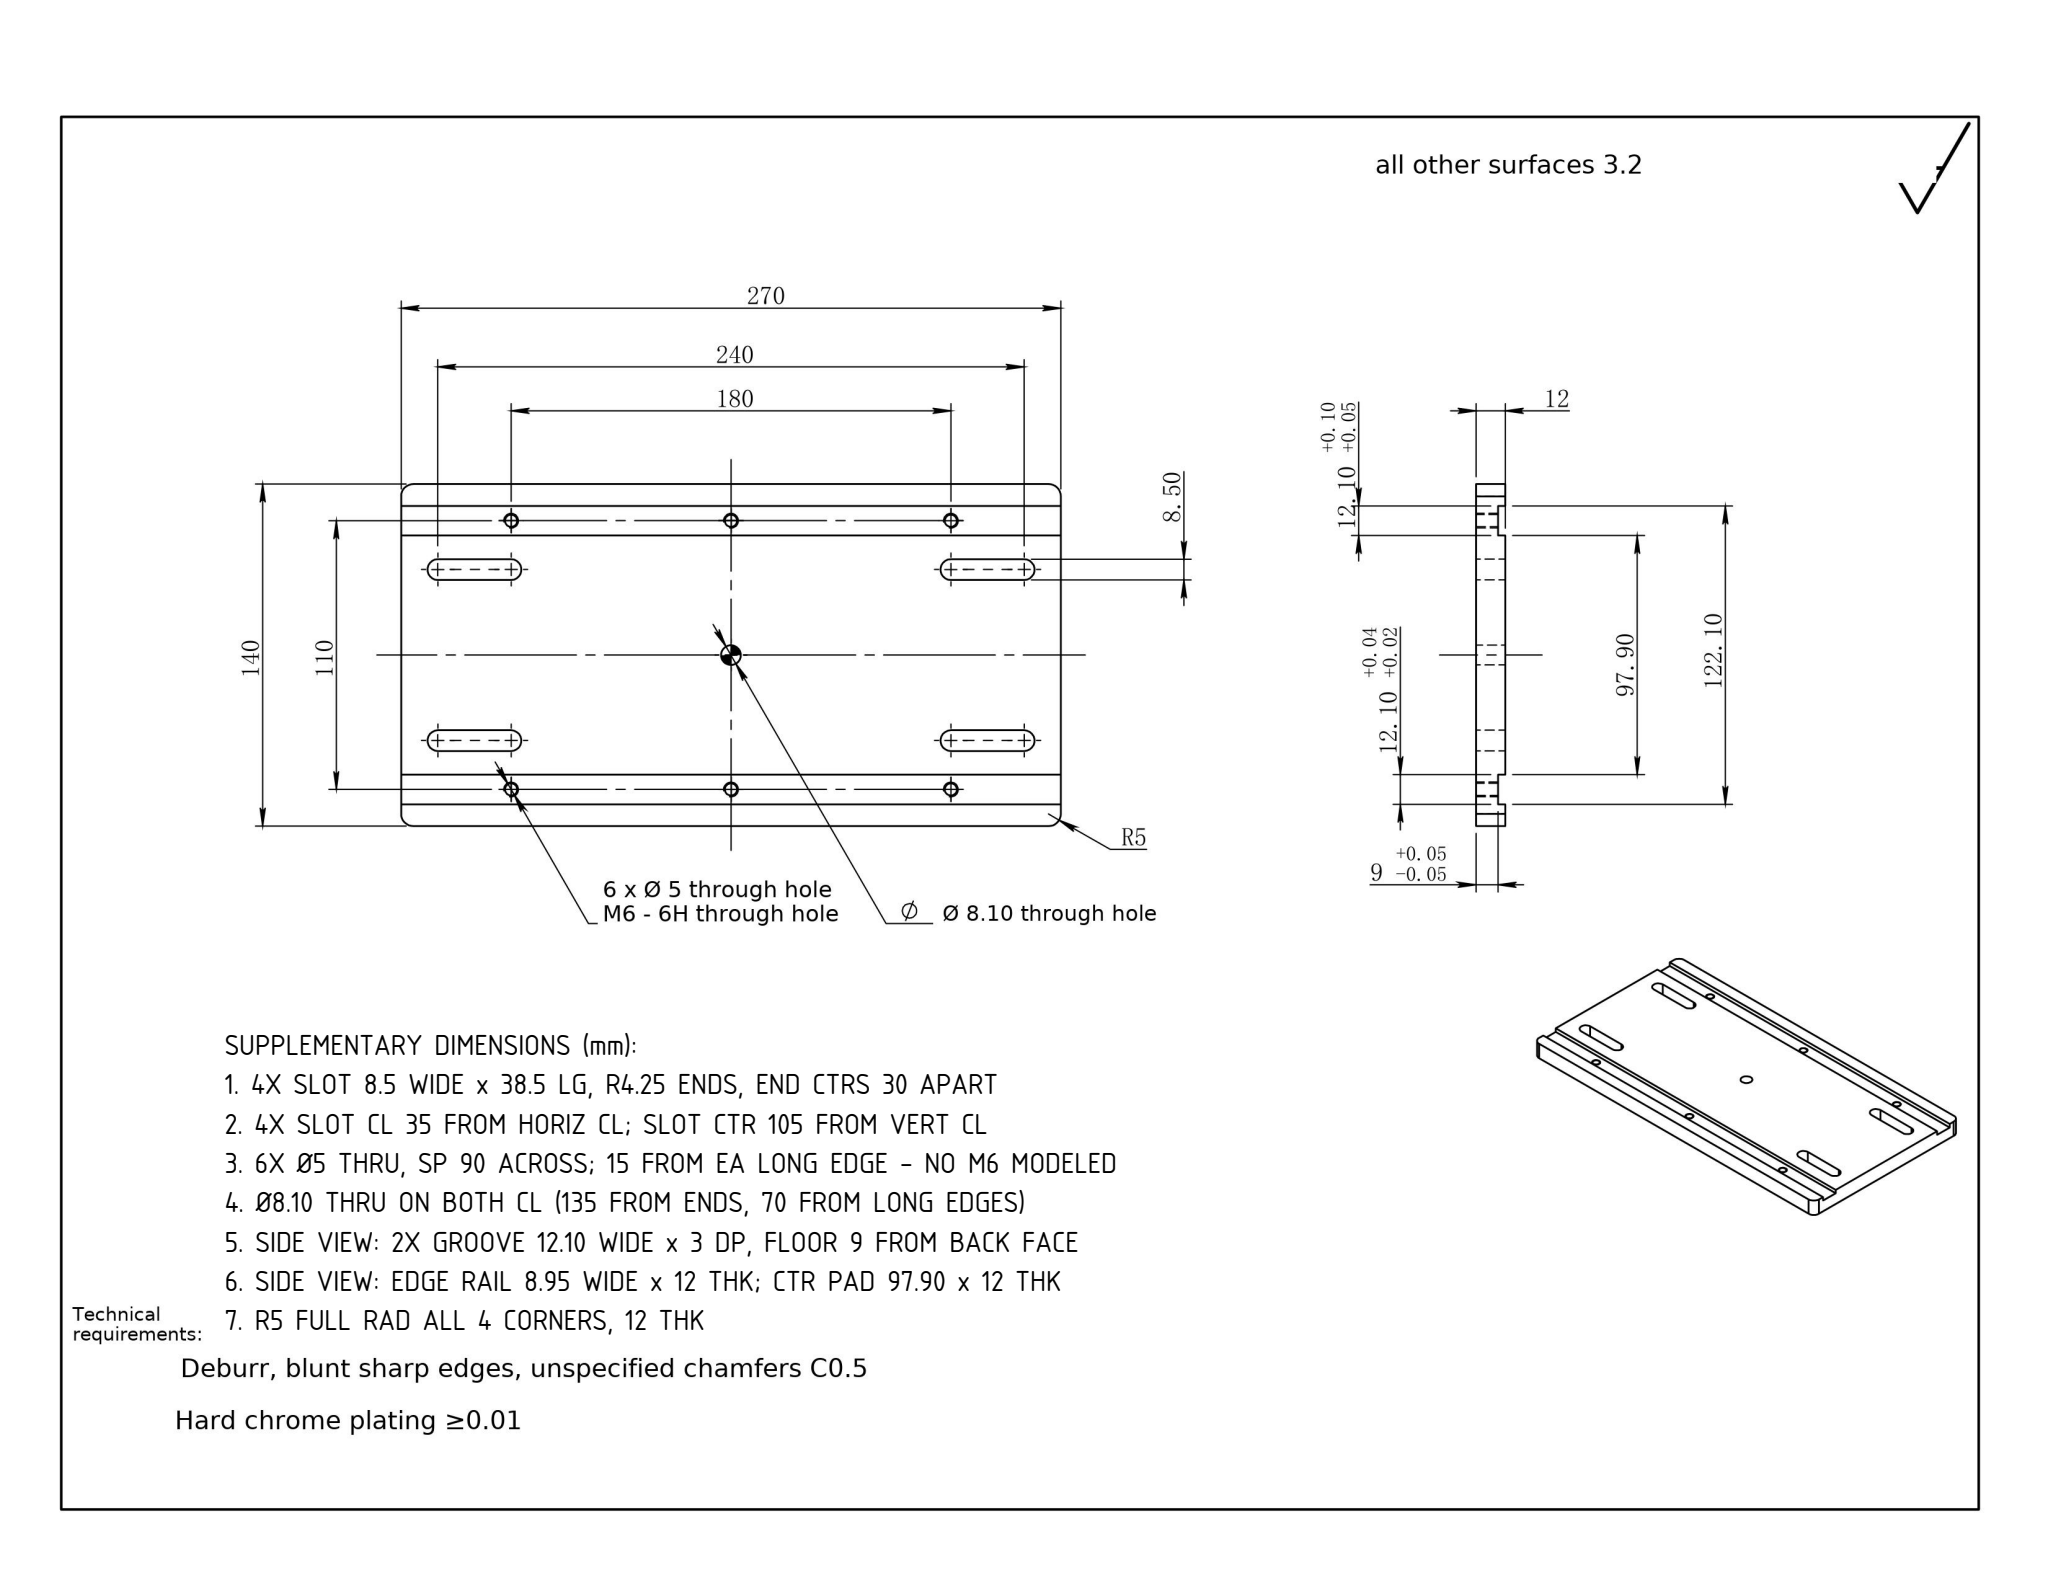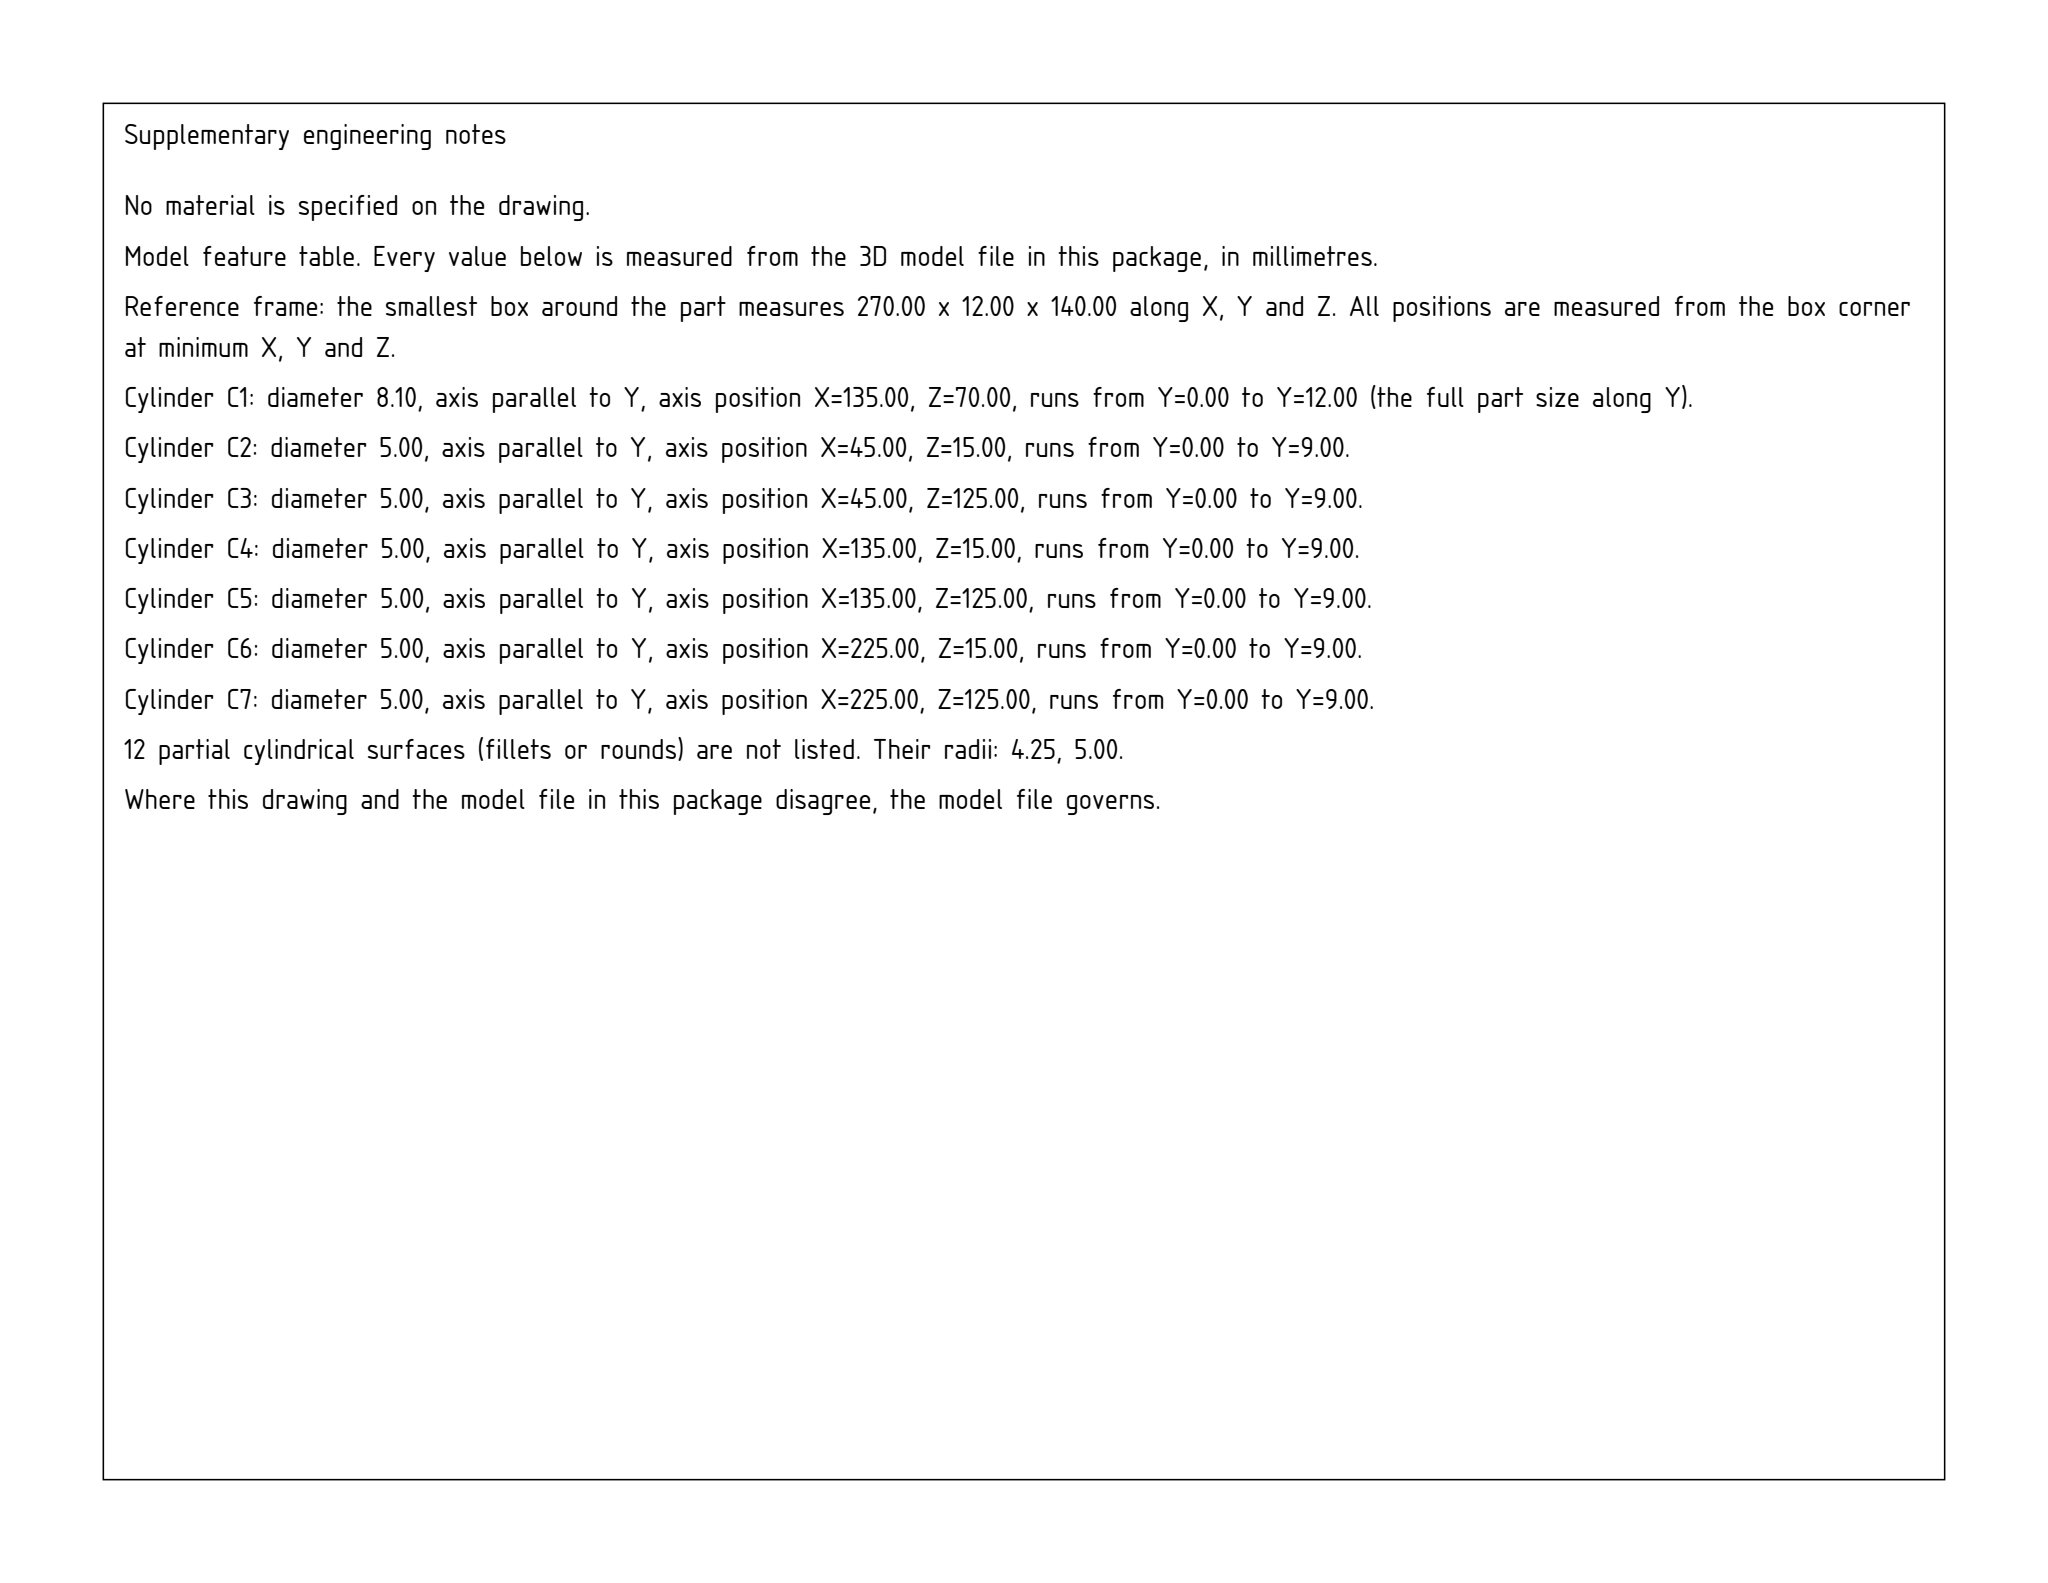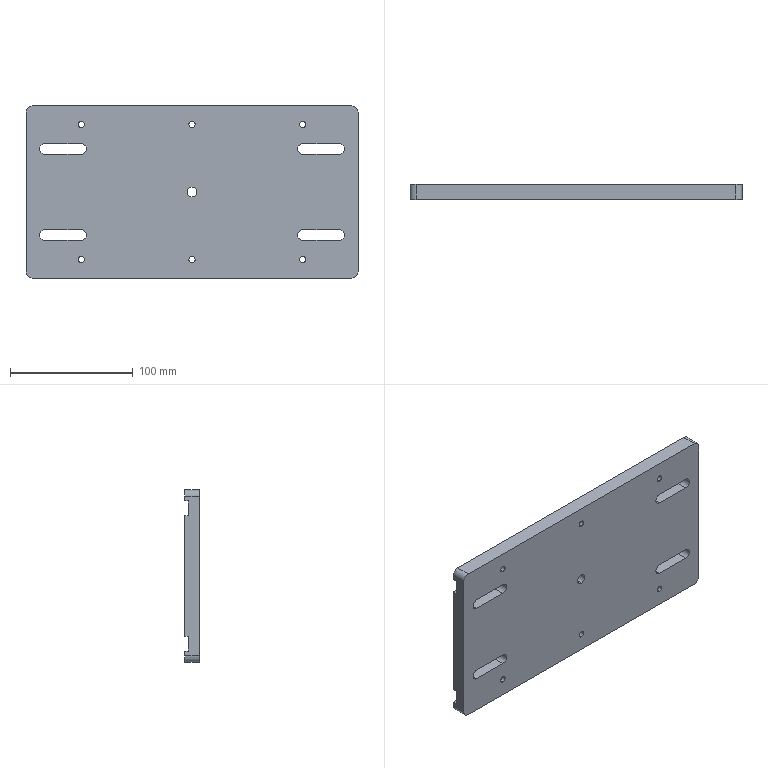Part | SolidWorks | mm | 1 solid | 48 faces | box 270 x 12 x 140 mm | volume 417098 mm3 | cylinder 26 | plane 22 | commonest cylinder face diameters 5 x12 8.5 x8 10 x4 8.1 x2
build123d program:
from build123d import *

# Parameters (mm, degrees)
SKETCH1_W                = 270
SKETCH1_H                = 140
BOSS_EXTRUDE1_DEPTH      = 12
SKETCH2_W                = 270
SKETCH2_H                = 12.1
CUT_EXTRUDE1_DEPTH       = 3
M6_TAPPED_HOLE1_D        = 5
LPATTERN1_COUNT          = 2
LPATTERN1_PITCH          = 90
LPATTERN1_COL_COUNT      = 2
LPATTERN1_COL_PITCH      = 90
FILLET1_R                = 5
F_8_0_8_DIAMETER_HOLE1_D = 8.1
CUT_EXTRUDE3_DEPTH       = 153.542


with BuildPart() as part:
    # Sketch1 → Boss-Extrude1 (new body)
    with BuildSketch(Plane(origin=(0, 0, 0), x_dir=(1, 0, 0), z_dir=(0, 1, 0))):
        Rectangle(SKETCH1_W, SKETCH1_H)
    extrude(amount=BOSS_EXTRUDE1_DEPTH)

    # Sketch2 → Cut-Extrude1 (cut)
    with BuildSketch(Plane(origin=(0, 12, 0), x_dir=(1, 0, 0), z_dir=(0, 1, 0))):
        with Locations((0, 55)):
            Rectangle(SKETCH2_W, SKETCH2_H)
        with Locations((0, -55)):
            Rectangle(SKETCH2_W, SKETCH2_H)
    extrude(amount=-CUT_EXTRUDE1_DEPTH, mode=Mode.SUBTRACT)

    # M6 Tapped Hole1 (through all)
    with Locations(Plane(origin=(0, 9, 0), x_dir=(1, 0, 0), z_dir=(0, 1, 0))):
        with Locations((0, -55), (0, 55)):
            m6_tapped_hole1 = Hole(M6_TAPPED_HOLE1_D / 2)

    # LPattern1: M6 Tapped Hole1 ×2
    with Locations(*[(i * LPATTERN1_PITCH, 0, 0) for i in range(1, LPATTERN1_COUNT)]):
        add(m6_tapped_hole1, mode=Mode.SUBTRACT)

    # LPattern1 col: M6 Tapped Hole1 ×2
    with Locations(*[(-i * LPATTERN1_COL_PITCH, 0, 0) for i in range(1, LPATTERN1_COL_COUNT)]):
        add(m6_tapped_hole1, mode=Mode.SUBTRACT)

    # Fillet1
    fillet1_edges = [part.edges().sort_by_distance(p)[0] for p in [
        (135, 6, 70),
        (-135, 6, 70),
        (-135, 6, -70),
        (135, 6, -70),
    ]]
    fillet(fillet1_edges, radius=FILLET1_R)

    # 8.0 _8_ Diameter Hole1 (through all)
    with Locations(Plane(origin=(0, 12, 0), x_dir=(1, 0, 0), z_dir=(0, 1, 0))):
        with Locations((0, 0)):
            Hole(F_8_0_8_DIAMETER_HOLE1_D / 2)

    # Sketch10 → Cut-Extrude3 (cut, through all)
    with BuildSketch(Plane(origin=(0, 12, 0), x_dir=(1, 0, 0), z_dir=(0, 1, 0))):
        with BuildLine():
            Line((-120, 39.25), (-90, 39.25))
            ThreePointArc((-90, 39.25), (-85.75, 35), (-90, 30.75))
            Line((-90, 30.75), (-120, 30.75))
            ThreePointArc((-120, 30.75), (-124.25, 35), (-120, 39.25))
        make_face()
        with BuildLine():
            Line((90, 39.25), (120, 39.25))
            ThreePointArc((120, 39.25), (124.25, 35), (120, 30.75))
            Line((120, 30.75), (90, 30.75))
            ThreePointArc((90, 30.75), (85.75, 35), (90, 39.25))
        make_face()
    cut_extrude3 = extrude(amount=-CUT_EXTRUDE3_DEPTH, mode=Mode.SUBTRACT)

    # Mirror1: Cut-Extrude3 across plane
    add(cut_extrude3.mirror(Plane.XY), mode=Mode.SUBTRACT)


solid = part.part